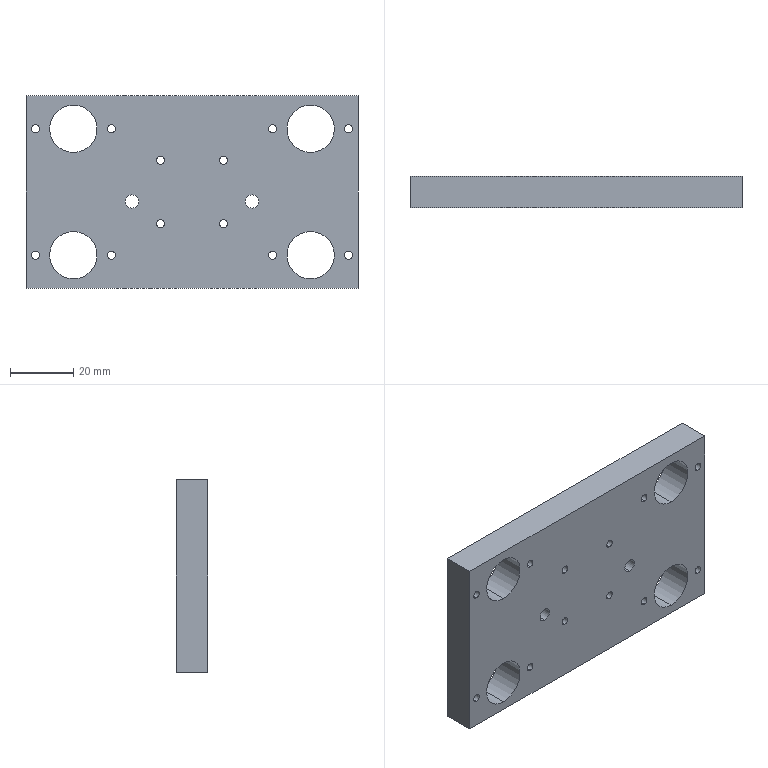Component | SolidWorks | F12529-M5103-1 | 1 solid | 42 faces | box 105 x 10 x 61 mm | volume 56115 mm3 | cylinder 36 | plane 6 | commonest cylinder face diameters 2.5 x24 15 x8 4.2 x4
build123d program:
from build123d import *

# Parameters (mm, degrees)
SKETCH1_W             = 105
SKETCH1_H             = 61
EXTRUDE1_DEPTH        = 10
SKETCH3_R             = 7.5
CUT_EXTRUDE1_DEPTH    = 62.535
M3_TAPPED_HOLE1_D     = 2.5
M3_TAPPED_HOLE2_D     = 2.5
MIRROR4_COPY_1_D      = 2.5
M5_TAPPED_HOLE1_D     = 4.2
M5_TAPPED_HOLE1_DEPTH = 12.4
M5_TAPPED_HOLE1_TIP   = 1.262


with BuildPart() as part:
    # Sketch1 → Extrude1 (new body)
    with BuildSketch(Plane(origin=(0, 0, 0), x_dir=(1, 0, 0), z_dir=(0, 1, 0))):
        Rectangle(SKETCH1_W, SKETCH1_H)
    extrude(amount=EXTRUDE1_DEPTH)

    # Sketch3 → Cut-Extrude1 (cut, through all)
    with BuildSketch(Plane(origin=(0, 10, 0), x_dir=(1, 0, 0), z_dir=(0, 1, 0))):
        with Locations(Location((37.5, 20, 0), (0, 0, 270))):
            Circle(SKETCH3_R)
        with Locations(Location((37.5, -20, 0), (0, 0, 270))):
            Circle(SKETCH3_R)
    cut_extrude1 = extrude(amount=-CUT_EXTRUDE1_DEPTH, mode=Mode.SUBTRACT)

    # Mirror1: Cut-Extrude1 across plane
    add(cut_extrude1.mirror(Plane(origin=(0, 0, 0), x_dir=(0, 0, 1), z_dir=(1, 0, 0))), mode=Mode.SUBTRACT)

    # M3 Tapped Hole1 (through all)
    with Locations(Plane(origin=(0, 10, 0), x_dir=(-1, 0, 0), z_dir=(0, 1, 0))):
        with Locations((-10, -10), (-10, 10)):
            m3_tapped_hole1 = Hole(M3_TAPPED_HOLE1_D / 2)

    # Mirror2: M3 Tapped Hole1 across plane
    add(m3_tapped_hole1.mirror(Plane(origin=(0, 0, 0), x_dir=(0, 0, 1), z_dir=(1, 0, 0))), mode=Mode.SUBTRACT)

    # M3 Tapped Hole2 (through all)
    with Locations(Plane.XZ):
        with Locations((49.5, 20), (25.5, 20)):
            m3_tapped_hole2 = Hole(M3_TAPPED_HOLE2_D / 2)

    # Mirror3: M3 Tapped Hole2 across plane
    add(m3_tapped_hole2.mirror(Plane.XY), mode=Mode.SUBTRACT)

    # Mirror4: M3 Tapped Hole2 across plane
    add(m3_tapped_hole2.mirror(Plane(origin=(0, 0, 0), x_dir=(0, 0, 1), z_dir=(1, 0, 0))), mode=Mode.SUBTRACT)

    # Mirror4 copy 1 (through all)
    with Locations(Plane(origin=(0, 0, 0), x_dir=(-1, 0, 0), z_dir=(0, -1, 0))):
        with Locations((49.5, 20), (25.5, 20)):
            Hole(MIRROR4_COPY_1_D / 2)

    # M5 Tapped Hole1
    with Locations(Plane(origin=(0, 10, 0), x_dir=(-1, 0, 0), z_dir=(0, 1, 0))):
        with Locations((-19, -3), (19, -3)):
            Hole(M5_TAPPED_HOLE1_D / 2, depth=M5_TAPPED_HOLE1_DEPTH)
            with Locations((0, 0, -(M5_TAPPED_HOLE1_DEPTH + M5_TAPPED_HOLE1_TIP / 2))):  # 118° drill point
                Cone(0, M5_TAPPED_HOLE1_D / 2, M5_TAPPED_HOLE1_TIP, mode=Mode.SUBTRACT)


solid = part.part

# Placed as in the assembly
solid = solid.moved(Location((0, 121, 0), (0, 0, 0)))